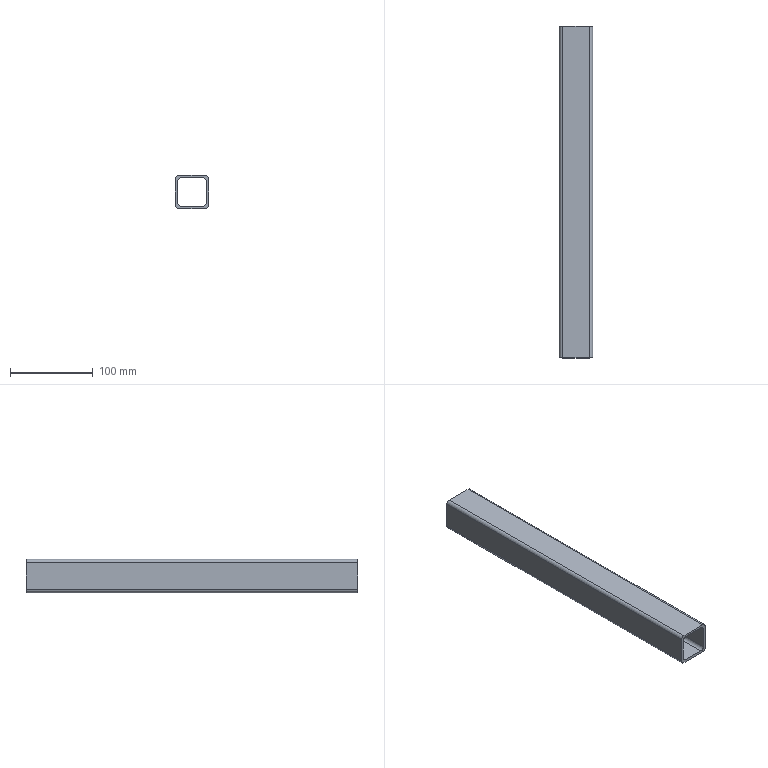Component | NX | SHORT_BOT_ROD_2 | 1 solid | 18 faces | volume 177600 mm3 | plane 10 | cylinder 8 | commonest cylinder face diameters 8 x8